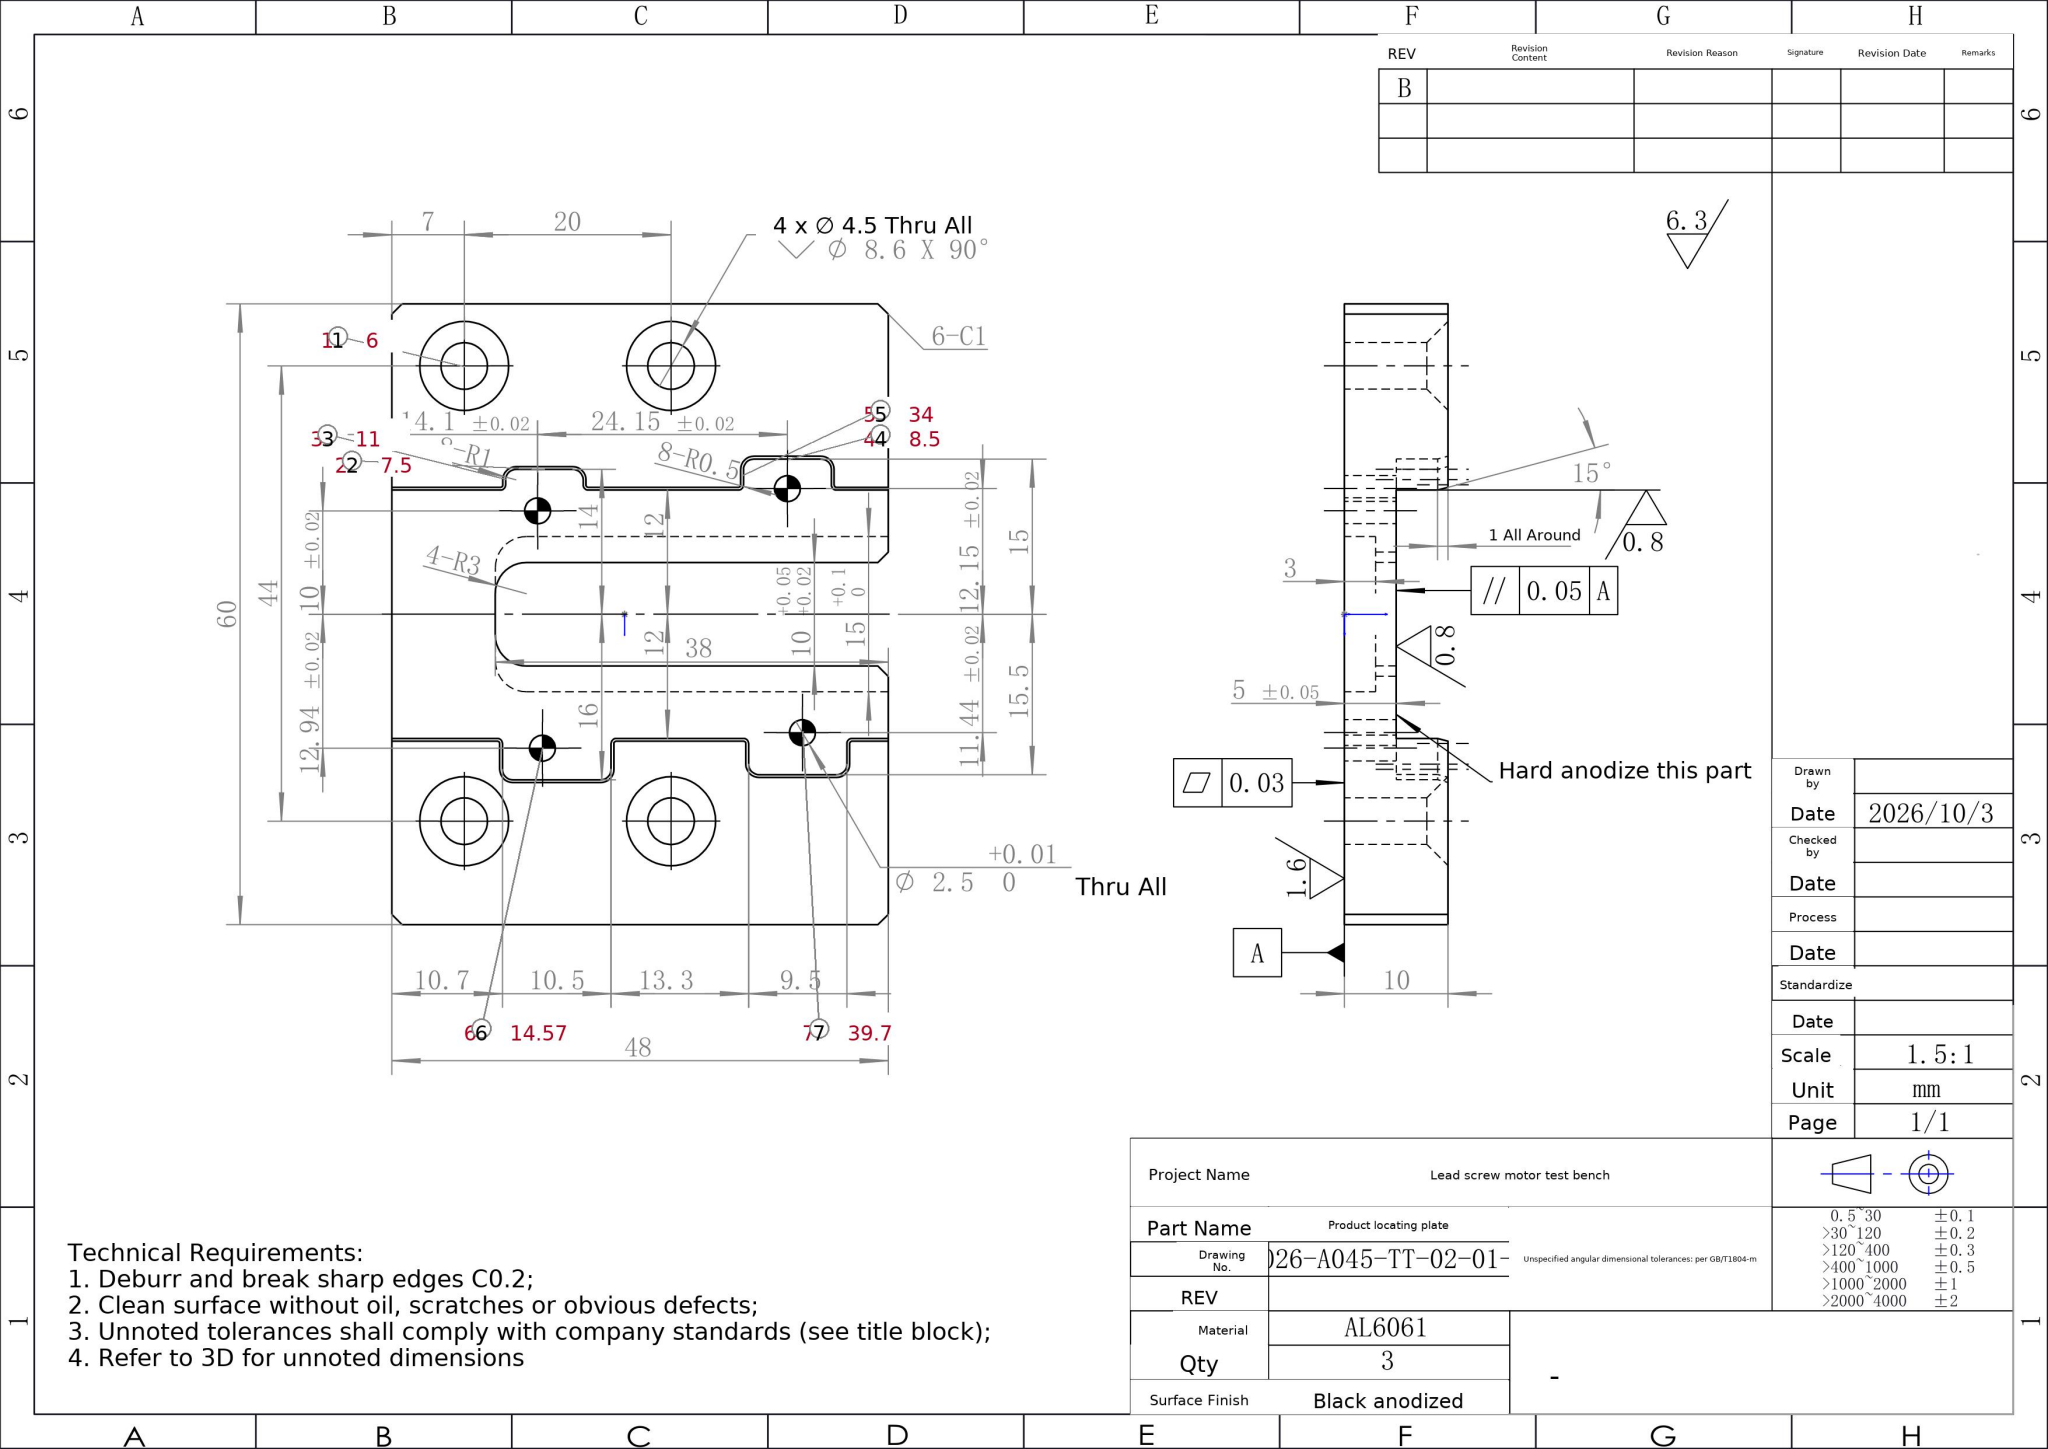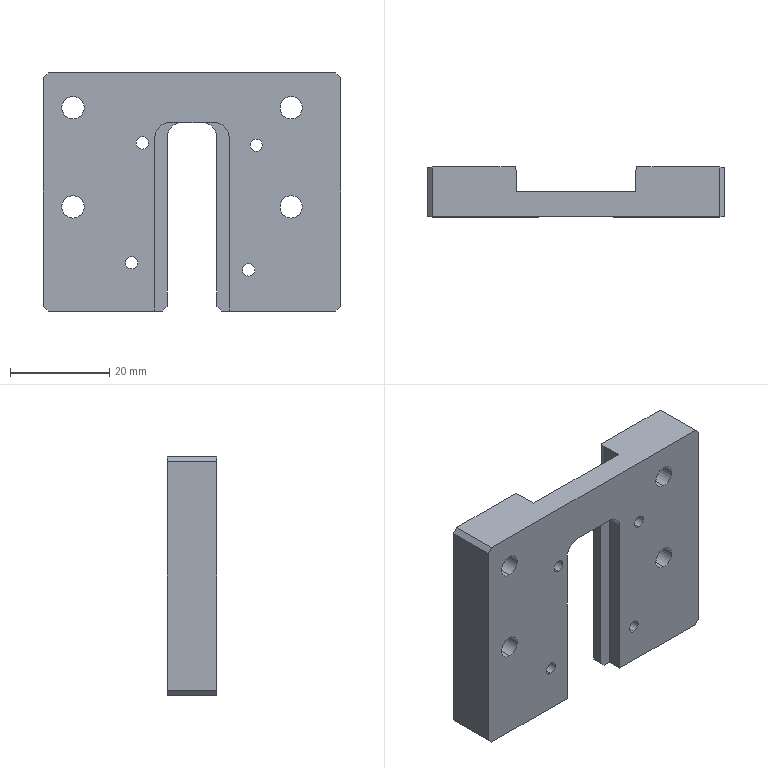Part | SolidWorks | mm | material AL6061 | 1 solid | 118 faces | box 60 x 10 x 48 mm | volume 19090 mm3 | plane 58 | cylinder 36 | cone 24 | commonest cylinder face diameters 2.5 x8 4.5 x8 2 x8 1 x8 6 x4